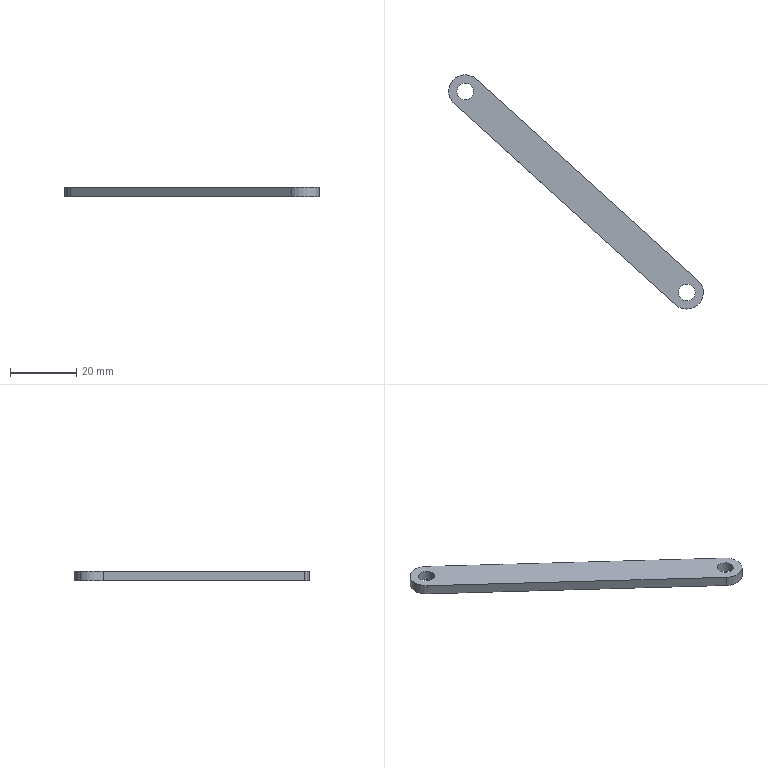Component | SolidWorks | WheelAssembly-1_ConnectingRod-1 | 1 solid | 11 faces | box 76.66 x 70.47 x 3 mm | volume 2818 mm3 | cylinder 7 | plane 4 | commonest cylinder face diameters 5 x4 10 x3
build123d program:
from build123d import *

# Parameters (mm, degrees)
SKETCH1_R           = 2.5
BOSS_EXTRUDE1_DEPTH = 3


with BuildPart() as part:
    # Sketch1 → Boss-Extrude1 (new body)
    with BuildSketch(Plane.XY):
        with BuildLine():
            Line((-45, 5), (45, 5))
            ThreePointArc((45, 5), (50, 0), (45, -5))
            Line((45, -5), (-45, -5))
            ThreePointArc((-45, -5), (-50, 0), (-45, 5))
        make_face()
        with Locations((-45, 0)):
            Circle(SKETCH1_R, mode=Mode.SUBTRACT)
        with Locations((45, 0)):
            Circle(SKETCH1_R, mode=Mode.SUBTRACT)
    extrude(amount=BOSS_EXTRUDE1_DEPTH)


solid = part.part

# Placed as in the assembly
solid = solid.moved(Location((-271.672, -91.236, -512.97), (0, 0, -42.215)))
STEP:
#1=COLOUR_RGB('',0.7922,0.8196,0.9333);
#2=FILL_AREA_STYLE_COLOUR('',#1);
#3=FILL_AREA_STYLE('',(#2));
#4=SURFACE_STYLE_FILL_AREA(#3);
#5=SURFACE_SIDE_STYLE('',(#4));
#6=SURFACE_STYLE_USAGE(.BOTH.,#5);
#7=PRESENTATION_STYLE_ASSIGNMENT((#6));
#8=CARTESIAN_POINT('',(-9.456,-4.716,-20.196));
#9=VERTEX_POINT('',#8);
#10=CARTESIAN_POINT('',(-9.311,-4.849,-20.196));
#11=VERTEX_POINT('',#10);
#12=CARTESIAN_POINT('',(-9.384,-4.782,-20.196));
#13=DIRECTION('',(-0.,-0.,-1.));
#14=DIRECTION('',(0.7406,-0.6719,0.));
#15=AXIS2_PLACEMENT_3D('',#12,#13,#14);
#16=CIRCLE('',#15,0.09843);
#17=EDGE_CURVE('',#9,#11,#16,.T.);
#18=ORIENTED_EDGE('',*,*,#17,.T.);
#19=CARTESIAN_POINT('',(-9.311,-4.849,-20.078));
#20=VERTEX_POINT('',#19);
#21=CARTESIAN_POINT('',(-9.311,-4.849,-20.196));
#22=DIRECTION('',(0.,0.,1.));
#23=VECTOR('',#22,39.37);
#24=LINE('',#21,#23);
#25=EDGE_CURVE('',#11,#20,#24,.T.);
#26=ORIENTED_EDGE('',*,*,#25,.T.);
#27=CARTESIAN_POINT('',(-9.456,-4.716,-20.078));
#28=VERTEX_POINT('',#27);
#29=CARTESIAN_POINT('',(-9.384,-4.782,-20.078));
#30=DIRECTION('',(-0.,-0.,-1.));
#31=DIRECTION('',(0.7406,-0.6719,0.));
#32=AXIS2_PLACEMENT_3D('',#29,#30,#31);
#33=CIRCLE('',#32,0.09843);
#34=EDGE_CURVE('',#28,#20,#33,.T.);
#35=ORIENTED_EDGE('',*,*,#34,.F.);
#36=CARTESIAN_POINT('',(-9.456,-4.716,-20.196));
#37=DIRECTION('',(0.,0.,1.));
#38=VECTOR('',#37,39.37);
#39=LINE('',#36,#38);
#40=EDGE_CURVE('',#9,#28,#39,.T.);
#41=ORIENTED_EDGE('',*,*,#40,.F.);
#42=EDGE_LOOP('',(#18,#26,#35,#41));
#43=FACE_OUTER_BOUND('',#42,.T.);
#44=CARTESIAN_POINT('',(-9.384,-4.782,-20.196));
#45=DIRECTION('',(0.,0.,1.));
#46=DIRECTION('',(-0.7406,0.6719,0.));
#47=AXIS2_PLACEMENT_3D('',#44,#45,#46);
#48=CYLINDRICAL_SURFACE('',#47,0.09843);
#49=ADVANCED_FACE('',(#43),#48,.F.);
#50=CARTESIAN_POINT('',(-12.081,-2.335,-20.196));
#51=VERTEX_POINT('',#50);
#52=CARTESIAN_POINT('',(-11.935,-2.468,-20.196));
#53=VERTEX_POINT('',#52);
#54=CARTESIAN_POINT('',(-12.008,-2.402,-20.196));
#55=DIRECTION('',(-0.,-0.,-1.));
#56=DIRECTION('',(0.7406,-0.6719,0.));
#57=AXIS2_PLACEMENT_3D('',#54,#55,#56);
#58=CIRCLE('',#57,0.09843);
#59=EDGE_CURVE('',#51,#53,#58,.T.);
#60=ORIENTED_EDGE('',*,*,#59,.T.);
#61=CARTESIAN_POINT('',(-11.935,-2.468,-20.078));
#62=VERTEX_POINT('',#61);
#63=CARTESIAN_POINT('',(-11.935,-2.468,-20.196));
#64=DIRECTION('',(0.,0.,1.));
#65=VECTOR('',#64,39.37);
#66=LINE('',#63,#65);
#67=EDGE_CURVE('',#53,#62,#66,.T.);
#68=ORIENTED_EDGE('',*,*,#67,.T.);
#69=CARTESIAN_POINT('',(-12.081,-2.335,-20.078));
#70=VERTEX_POINT('',#69);
#71=CARTESIAN_POINT('',(-12.008,-2.402,-20.078));
#72=DIRECTION('',(-0.,-0.,-1.));
#73=DIRECTION('',(0.7406,-0.6719,0.));
#74=AXIS2_PLACEMENT_3D('',#71,#72,#73);
#75=CIRCLE('',#74,0.09843);
#76=EDGE_CURVE('',#70,#62,#75,.T.);
#77=ORIENTED_EDGE('',*,*,#76,.F.);
#78=CARTESIAN_POINT('',(-12.081,-2.335,-20.196));
#79=DIRECTION('',(0.,0.,1.));
#80=VECTOR('',#79,39.37);
#81=LINE('',#78,#80);
#82=EDGE_CURVE('',#51,#70,#81,.T.);
#83=ORIENTED_EDGE('',*,*,#82,.F.);
#84=EDGE_LOOP('',(#60,#68,#77,#83));
#85=FACE_OUTER_BOUND('',#84,.T.);
#86=CARTESIAN_POINT('',(-12.008,-2.402,-20.196));
#87=DIRECTION('',(0.,0.,1.));
#88=DIRECTION('',(-0.7406,0.6719,0.));
#89=AXIS2_PLACEMENT_3D('',#86,#87,#88);
#90=CYLINDRICAL_SURFACE('',#89,0.09843);
#91=ADVANCED_FACE('',(#85),#90,.F.);
#92=CARTESIAN_POINT('',(-12.154,-2.269,-20.196));
#93=VERTEX_POINT('',#92);
#94=CARTESIAN_POINT('',(-11.876,-2.256,-20.196));
#95=VERTEX_POINT('',#94);
#96=CARTESIAN_POINT('',(-12.008,-2.402,-20.196));
#97=DIRECTION('',(-0.,-0.,-1.));
#98=DIRECTION('',(0.7406,-0.6719,0.));
#99=AXIS2_PLACEMENT_3D('',#96,#97,#98);
#100=CIRCLE('',#99,0.1969);
#101=EDGE_CURVE('',#93,#95,#100,.T.);
#102=ORIENTED_EDGE('',*,*,#101,.F.);
#103=CARTESIAN_POINT('',(-12.154,-2.269,-20.078));
#104=VERTEX_POINT('',#103);
#105=CARTESIAN_POINT('',(-12.154,-2.269,-20.196));
#106=DIRECTION('',(0.,0.,1.));
#107=VECTOR('',#106,39.37);
#108=LINE('',#105,#107);
#109=EDGE_CURVE('',#93,#104,#108,.T.);
#110=ORIENTED_EDGE('',*,*,#109,.T.);
#111=CARTESIAN_POINT('',(-11.876,-2.256,-20.078));
#112=VERTEX_POINT('',#111);
#113=CARTESIAN_POINT('',(-12.008,-2.402,-20.078));
#114=DIRECTION('',(-0.,-0.,-1.));
#115=DIRECTION('',(0.7406,-0.6719,0.));
#116=AXIS2_PLACEMENT_3D('',#113,#114,#115);
#117=CIRCLE('',#116,0.1969);
#118=EDGE_CURVE('',#104,#112,#117,.T.);
#119=ORIENTED_EDGE('',*,*,#118,.T.);
#120=CARTESIAN_POINT('',(-11.876,-2.256,-20.196));
#121=DIRECTION('',(0.,0.,1.));
#122=VECTOR('',#121,39.37);
#123=LINE('',#120,#122);
#124=EDGE_CURVE('',#95,#112,#123,.T.);
#125=ORIENTED_EDGE('',*,*,#124,.F.);
#126=EDGE_LOOP('',(#102,#110,#119,#125));
#127=FACE_OUTER_BOUND('',#126,.T.);
#128=CARTESIAN_POINT('',(-12.008,-2.402,-20.196));
#129=DIRECTION('',(0.,0.,1.));
#130=DIRECTION('',(-0.7406,0.6719,0.));
#131=AXIS2_PLACEMENT_3D('',#128,#129,#130);
#132=CYLINDRICAL_SURFACE('',#131,0.1969);
#133=ADVANCED_FACE('',(#127),#132,.T.);
#134=ORIENTED_EDGE('',*,*,#59,.F.);
#135=CARTESIAN_POINT('',(-12.008,-2.402,-20.196));
#136=DIRECTION('',(-0.,-0.,-1.));
#137=DIRECTION('',(0.7406,-0.6719,0.));
#138=AXIS2_PLACEMENT_3D('',#135,#136,#137);
#139=CIRCLE('',#138,0.09843);
#140=EDGE_CURVE('',#53,#51,#139,.T.);
#141=ORIENTED_EDGE('',*,*,#140,.F.);
#142=EDGE_LOOP('',(#134,#141));
#143=FACE_BOUND('',#142,.T.);
#144=CARTESIAN_POINT('',(-12.14,-2.547,-20.196));
#145=VERTEX_POINT('',#144);
#146=CARTESIAN_POINT('',(-12.008,-2.402,-20.196));
#147=DIRECTION('',(-0.,-0.,-1.));
#148=DIRECTION('',(0.7406,-0.6719,0.));
#149=AXIS2_PLACEMENT_3D('',#146,#147,#148);
#150=CIRCLE('',#149,0.1969);
#151=EDGE_CURVE('',#145,#93,#150,.T.);
#152=ORIENTED_EDGE('',*,*,#151,.T.);
#153=ORIENTED_EDGE('',*,*,#101,.T.);
#154=CARTESIAN_POINT('',(-9.251,-4.637,-20.196));
#155=VERTEX_POINT('',#154);
#156=CARTESIAN_POINT('',(-11.876,-2.256,-20.196));
#157=DIRECTION('',(0.7406,-0.6719,0.));
#158=VECTOR('',#157,39.37);
#159=LINE('',#156,#158);
#160=EDGE_CURVE('',#95,#155,#159,.T.);
#161=ORIENTED_EDGE('',*,*,#160,.T.);
#162=CARTESIAN_POINT('',(-9.516,-4.928,-20.196));
#163=VERTEX_POINT('',#162);
#164=CARTESIAN_POINT('',(-9.384,-4.782,-20.196));
#165=DIRECTION('',(-0.,-0.,-1.));
#166=DIRECTION('',(0.7406,-0.6719,0.));
#167=AXIS2_PLACEMENT_3D('',#164,#165,#166);
#168=CIRCLE('',#167,0.1969);
#169=EDGE_CURVE('',#155,#163,#168,.T.);
#170=ORIENTED_EDGE('',*,*,#169,.T.);
#171=CARTESIAN_POINT('',(-12.14,-2.547,-20.196));
#172=DIRECTION('',(-0.7406,0.6719,-0.));
#173=VECTOR('',#172,39.37);
#174=LINE('',#171,#173);
#175=EDGE_CURVE('',#163,#145,#174,.T.);
#176=ORIENTED_EDGE('',*,*,#175,.T.);
#177=EDGE_LOOP('',(#152,#153,#161,#170,#176));
#178=FACE_OUTER_BOUND('',#177,.T.);
#179=ORIENTED_EDGE('',*,*,#17,.F.);
#180=CARTESIAN_POINT('',(-9.384,-4.782,-20.196));
#181=DIRECTION('',(-0.,-0.,-1.));
#182=DIRECTION('',(0.7406,-0.6719,0.));
#183=AXIS2_PLACEMENT_3D('',#180,#181,#182);
#184=CIRCLE('',#183,0.09843);
#185=EDGE_CURVE('',#11,#9,#184,.T.);
#186=ORIENTED_EDGE('',*,*,#185,.F.);
#187=EDGE_LOOP('',(#179,#186));
#188=FACE_BOUND('',#187,.T.);
#189=CARTESIAN_POINT('',(-12.008,-2.402,-20.196));
#190=DIRECTION('',(-0.,-0.,-1.));
#191=DIRECTION('',(0.7406,-0.6719,0.));
#192=AXIS2_PLACEMENT_3D('',#189,#190,#191);
#193=PLANE('',#192);
#194=ADVANCED_FACE('',(#143,#178,#188),#193,.T.);
#195=CARTESIAN_POINT('',(-12.14,-2.547,-20.078));
#196=VERTEX_POINT('',#195);
#197=CARTESIAN_POINT('',(-12.008,-2.402,-20.078));
#198=DIRECTION('',(-0.,-0.,-1.));
#199=DIRECTION('',(0.7406,-0.6719,0.));
#200=AXIS2_PLACEMENT_3D('',#197,#198,#199);
#201=CIRCLE('',#200,0.1969);
#202=EDGE_CURVE('',#196,#104,#201,.T.);
#203=ORIENTED_EDGE('',*,*,#202,.F.);
#204=CARTESIAN_POINT('',(-9.516,-4.928,-20.078));
#205=VERTEX_POINT('',#204);
#206=CARTESIAN_POINT('',(-12.14,-2.547,-20.078));
#207=DIRECTION('',(-0.7406,0.6719,-0.));
#208=VECTOR('',#207,39.37);
#209=LINE('',#206,#208);
#210=EDGE_CURVE('',#205,#196,#209,.T.);
#211=ORIENTED_EDGE('',*,*,#210,.F.);
#212=CARTESIAN_POINT('',(-9.251,-4.637,-20.078));
#213=VERTEX_POINT('',#212);
#214=CARTESIAN_POINT('',(-9.384,-4.782,-20.078));
#215=DIRECTION('',(-0.,-0.,-1.));
#216=DIRECTION('',(0.7406,-0.6719,0.));
#217=AXIS2_PLACEMENT_3D('',#214,#215,#216);
#218=CIRCLE('',#217,0.1969);
#219=EDGE_CURVE('',#213,#205,#218,.T.);
#220=ORIENTED_EDGE('',*,*,#219,.F.);
#221=CARTESIAN_POINT('',(-11.876,-2.256,-20.078));
#222=DIRECTION('',(0.7406,-0.6719,0.));
#223=VECTOR('',#222,39.37);
#224=LINE('',#221,#223);
#225=EDGE_CURVE('',#112,#213,#224,.T.);
#226=ORIENTED_EDGE('',*,*,#225,.F.);
#227=ORIENTED_EDGE('',*,*,#118,.F.);
#228=EDGE_LOOP('',(#203,#211,#220,#226,#227));
#229=FACE_OUTER_BOUND('',#228,.T.);
#230=ORIENTED_EDGE('',*,*,#76,.T.);
#231=CARTESIAN_POINT('',(-12.008,-2.402,-20.078));
#232=DIRECTION('',(-0.,-0.,-1.));
#233=DIRECTION('',(0.7406,-0.6719,0.));
#234=AXIS2_PLACEMENT_3D('',#231,#232,#233);
#235=CIRCLE('',#234,0.09843);
#236=EDGE_CURVE('',#62,#70,#235,.T.);
#237=ORIENTED_EDGE('',*,*,#236,.T.);
#238=EDGE_LOOP('',(#230,#237));
#239=FACE_BOUND('',#238,.T.);
#240=ORIENTED_EDGE('',*,*,#34,.T.);
#241=CARTESIAN_POINT('',(-9.384,-4.782,-20.078));
#242=DIRECTION('',(-0.,-0.,-1.));
#243=DIRECTION('',(0.7406,-0.6719,0.));
#244=AXIS2_PLACEMENT_3D('',#241,#242,#243);
#245=CIRCLE('',#244,0.09843);
#246=EDGE_CURVE('',#20,#28,#245,.T.);
#247=ORIENTED_EDGE('',*,*,#246,.T.);
#248=EDGE_LOOP('',(#240,#247));
#249=FACE_BOUND('',#248,.T.);
#250=CARTESIAN_POINT('',(-12.008,-2.402,-20.078));
#251=DIRECTION('',(-0.,-0.,-1.));
#252=DIRECTION('',(0.7406,-0.6719,0.));
#253=AXIS2_PLACEMENT_3D('',#250,#251,#252);
#254=PLANE('',#253);
#255=ADVANCED_FACE('',(#229,#239,#249),#254,.F.);
#256=ORIENTED_EDGE('',*,*,#109,.F.);
#257=ORIENTED_EDGE('',*,*,#151,.F.);
#258=CARTESIAN_POINT('',(-12.14,-2.547,-20.196));
#259=DIRECTION('',(0.,0.,1.));
#260=VECTOR('',#259,39.37);
#261=LINE('',#258,#260);
#262=EDGE_CURVE('',#145,#196,#261,.T.);
#263=ORIENTED_EDGE('',*,*,#262,.T.);
#264=ORIENTED_EDGE('',*,*,#202,.T.);
#265=EDGE_LOOP('',(#256,#257,#263,#264));
#266=FACE_OUTER_BOUND('',#265,.T.);
#267=CARTESIAN_POINT('',(-12.008,-2.402,-20.196));
#268=DIRECTION('',(0.,0.,1.));
#269=DIRECTION('',(-0.7406,0.6719,0.));
#270=AXIS2_PLACEMENT_3D('',#267,#268,#269);
#271=CYLINDRICAL_SURFACE('',#270,0.1969);
#272=ADVANCED_FACE('',(#266),#271,.T.);
#273=ORIENTED_EDGE('',*,*,#225,.T.);
#274=CARTESIAN_POINT('',(-9.251,-4.637,-20.196));
#275=DIRECTION('',(0.,0.,1.));
#276=VECTOR('',#275,39.37);
#277=LINE('',#274,#276);
#278=EDGE_CURVE('',#155,#213,#277,.T.);
#279=ORIENTED_EDGE('',*,*,#278,.F.);
#280=ORIENTED_EDGE('',*,*,#160,.F.);
#281=ORIENTED_EDGE('',*,*,#124,.T.);
#282=EDGE_LOOP('',(#273,#279,#280,#281));
#283=FACE_OUTER_BOUND('',#282,.T.);
#284=CARTESIAN_POINT('',(-11.876,-2.256,-20.196));
#285=DIRECTION('',(-0.6719,-0.7406,0.));
#286=DIRECTION('',(-0.,-0.,-1.));
#287=AXIS2_PLACEMENT_3D('',#284,#285,#286);
#288=PLANE('',#287);
#289=ADVANCED_FACE('',(#283),#288,.F.);
#290=ORIENTED_EDGE('',*,*,#219,.T.);
#291=CARTESIAN_POINT('',(-9.516,-4.928,-20.196));
#292=DIRECTION('',(0.,0.,1.));
#293=VECTOR('',#292,39.37);
#294=LINE('',#291,#293);
#295=EDGE_CURVE('',#163,#205,#294,.T.);
#296=ORIENTED_EDGE('',*,*,#295,.F.);
#297=ORIENTED_EDGE('',*,*,#169,.F.);
#298=ORIENTED_EDGE('',*,*,#278,.T.);
#299=EDGE_LOOP('',(#290,#296,#297,#298));
#300=FACE_OUTER_BOUND('',#299,.T.);
#301=CARTESIAN_POINT('',(-9.384,-4.782,-20.196));
#302=DIRECTION('',(0.,0.,1.));
#303=DIRECTION('',(-0.7406,0.6719,0.));
#304=AXIS2_PLACEMENT_3D('',#301,#302,#303);
#305=CYLINDRICAL_SURFACE('',#304,0.1969);
#306=ADVANCED_FACE('',(#300),#305,.T.);
#307=ORIENTED_EDGE('',*,*,#210,.T.);
#308=ORIENTED_EDGE('',*,*,#262,.F.);
#309=ORIENTED_EDGE('',*,*,#175,.F.);
#310=ORIENTED_EDGE('',*,*,#295,.T.);
#311=EDGE_LOOP('',(#307,#308,#309,#310));
#312=FACE_OUTER_BOUND('',#311,.T.);
#313=CARTESIAN_POINT('',(-12.14,-2.547,-20.196));
#314=DIRECTION('',(0.6719,0.7406,-0.));
#315=DIRECTION('',(0.7406,-0.6719,0.));
#316=AXIS2_PLACEMENT_3D('',#313,#314,#315);
#317=PLANE('',#316);
#318=ADVANCED_FACE('',(#312),#317,.F.);
#319=ORIENTED_EDGE('',*,*,#67,.F.);
#320=ORIENTED_EDGE('',*,*,#140,.T.);
#321=ORIENTED_EDGE('',*,*,#82,.T.);
#322=ORIENTED_EDGE('',*,*,#236,.F.);
#323=EDGE_LOOP('',(#319,#320,#321,#322));
#324=FACE_OUTER_BOUND('',#323,.T.);
#325=CARTESIAN_POINT('',(-12.008,-2.402,-20.196));
#326=DIRECTION('',(0.,0.,1.));
#327=DIRECTION('',(-0.7406,0.6719,0.));
#328=AXIS2_PLACEMENT_3D('',#325,#326,#327);
#329=CYLINDRICAL_SURFACE('',#328,0.09843);
#330=ADVANCED_FACE('',(#324),#329,.F.);
#331=ORIENTED_EDGE('',*,*,#25,.F.);
#332=ORIENTED_EDGE('',*,*,#185,.T.);
#333=ORIENTED_EDGE('',*,*,#40,.T.);
#334=ORIENTED_EDGE('',*,*,#246,.F.);
#335=EDGE_LOOP('',(#331,#332,#333,#334));
#336=FACE_OUTER_BOUND('',#335,.T.);
#337=CARTESIAN_POINT('',(-9.384,-4.782,-20.196));
#338=DIRECTION('',(0.,0.,1.));
#339=DIRECTION('',(-0.7406,0.6719,0.));
#340=AXIS2_PLACEMENT_3D('',#337,#338,#339);
#341=CYLINDRICAL_SURFACE('',#340,0.09843);
#342=ADVANCED_FACE('',(#336),#341,.F.);
#343=CLOSED_SHELL('',(#49,#91,#133,#194,#255,#272,#289,#306,#318,#330,#342));
#344=MANIFOLD_SOLID_BREP('',#343);
#345=STYLED_ITEM('',(#7),#344);
#346=(LENGTH_UNIT()NAMED_UNIT(*)SI_UNIT($,.METRE.));
#347=LENGTH_MEASURE_WITH_UNIT(LENGTH_MEASURE(0.0254),#346);
#348=DIMENSIONAL_EXPONENTS(1.,0.,0.,0.,0.,0.,0.);
#349=(CONVERSION_BASED_UNIT('',#347)LENGTH_UNIT()NAMED_UNIT(#348));
#350=UNCERTAINTY_MEASURE_WITH_UNIT(LENGTH_MEASURE(0.00001),#349,'','');
#351=(NAMED_UNIT(*)PLANE_ANGLE_UNIT()SI_UNIT($,.RADIAN.));
#352=(NAMED_UNIT(*)SI_UNIT($,.STERADIAN.)SOLID_ANGLE_UNIT());
#353=(GEOMETRIC_REPRESENTATION_CONTEXT(3)GLOBAL_UNCERTAINTY_ASSIGNED_CONTEXT((#350))GLOBAL_UNIT_ASSIGNED_CONTEXT((#349,#351,#352))REPRESENTATION_CONTEXT('',''));
#354=MECHANICAL_DESIGN_GEOMETRIC_PRESENTATION_REPRESENTATION('',(#345),#353);
#355=CARTESIAN_POINT('',(0.,0.,0.));
#356=DIRECTION('',(0.,0.,1.));
#357=DIRECTION('',(1.,0.,0.));
#358=AXIS2_PLACEMENT_3D('',#355,#356,#357);
#359=(LENGTH_UNIT()NAMED_UNIT(*)SI_UNIT($,.METRE.));
#360=LENGTH_MEASURE_WITH_UNIT(LENGTH_MEASURE(0.0254),#359);
#361=DIMENSIONAL_EXPONENTS(1.,0.,0.,0.,0.,0.,0.);
#362=(CONVERSION_BASED_UNIT('',#360)LENGTH_UNIT()NAMED_UNIT(#361));
#363=UNCERTAINTY_MEASURE_WITH_UNIT(LENGTH_MEASURE(0.00001),#362,'','');
#364=(NAMED_UNIT(*)PLANE_ANGLE_UNIT()SI_UNIT($,.RADIAN.));
#365=(NAMED_UNIT(*)SI_UNIT($,.STERADIAN.)SOLID_ANGLE_UNIT());
#366=(GEOMETRIC_REPRESENTATION_CONTEXT(3)GLOBAL_UNCERTAINTY_ASSIGNED_CONTEXT((#363))GLOBAL_UNIT_ASSIGNED_CONTEXT((#362,#364,#365))REPRESENTATION_CONTEXT('',''));
#367=ADVANCED_BREP_SHAPE_REPRESENTATION('',(#344,#358),#366);
#368=PRESENTATION_LAYER_ASSIGNMENT('','',(#345));